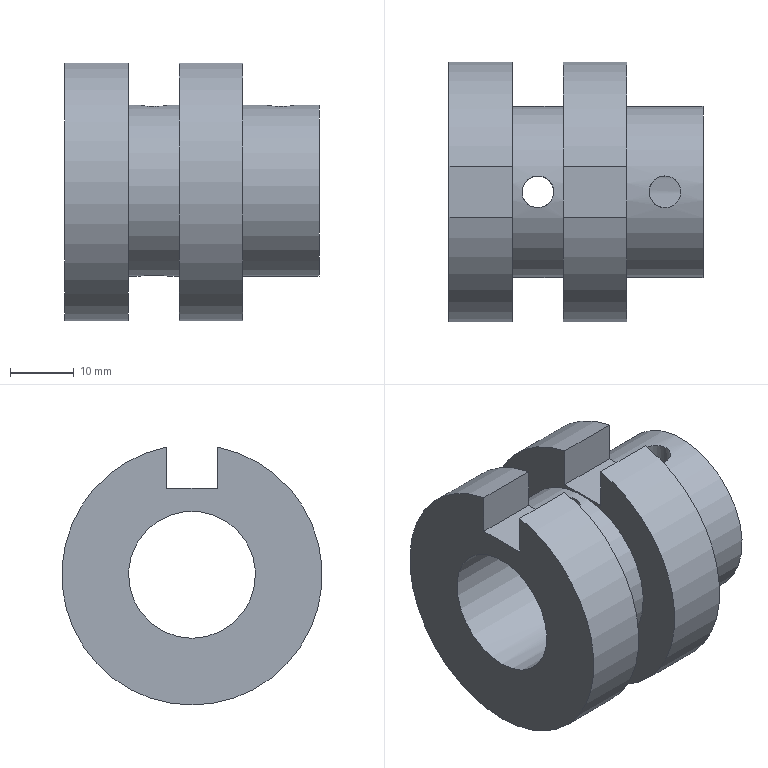Component | NX | STOP_BLOCK_WP | 1 solid | 19 faces | volume 24000 mm3 | plane 11 | cylinder 8 | commonest cylinder face diameters 5 x3 27 x2 41 x2 20 x1